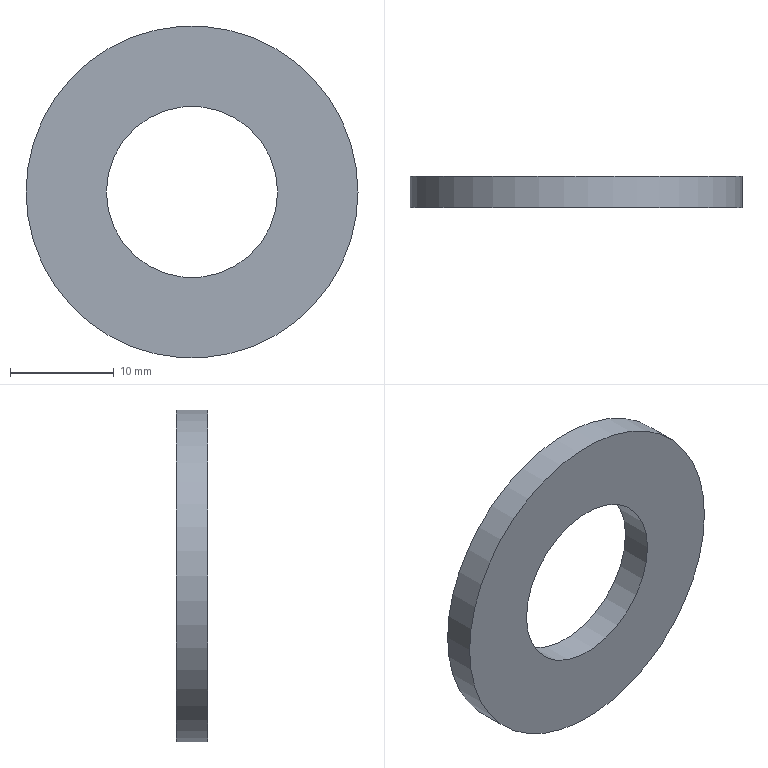Component | NX | WASHER | 1 solid | 4 faces | box 32 x 3 x 32 mm | volume 1771 mm3 | cylinder 2 | plane 2 | commonest cylinder face diameters 32 x1 16.5 x1
STEP:
#1=CARTESIAN_POINT('',(0.,0.,0.));
#2=DIRECTION('',(0.,0.,1.));
#3=DIRECTION('',(1.,0.,0.));
#4=AXIS2_PLACEMENT_3D('',#1,#2,#3);
#5=CARTESIAN_POINT('',(-1.,48.,105.));
#6=VERTEX_POINT('',#5);
#7=CARTESIAN_POINT('',(-17.,48.,105.));
#8=DIRECTION('',(0.,-1.,0.));
#9=DIRECTION('',(1.,0.,0.));
#10=AXIS2_PLACEMENT_3D('',#7,#8,#9);
#11=CIRCLE('',#10,16.);
#12=CARTESIAN_POINT('',(-17.,48.,105.));
#13=DIRECTION('',(0.,-1.,0.));
#14=DIRECTION('',(0.,0.,-1.));
#15=AXIS2_PLACEMENT_3D('',#12,#13,#14);
#16=CYLINDRICAL_SURFACE('',#15,16.);
#17=CARTESIAN_POINT('',(1.571,0.));
#18=DIRECTION('',(1.,0.));
#19=VECTOR('',#18,1.);
#20=LINE('',#17,#19);
#21=(GEOMETRIC_REPRESENTATION_CONTEXT(2)PARAMETRIC_REPRESENTATION_CONTEXT()REPRESENTATION_CONTEXT('',''));
#22=DEFINITIONAL_REPRESENTATION('',(#20),#21);
#23=PCURVE('',#16,#22);
#24=CARTESIAN_POINT('',(-17.,48.,105.));
#25=DIRECTION('',(0.,-1.,0.));
#26=DIRECTION('',(0.,0.,-1.));
#27=AXIS2_PLACEMENT_3D('',#24,#25,#26);
#28=PLANE('',#27);
#29=CARTESIAN_POINT('',(0.,0.));
#30=DIRECTION('',(0.,1.));
#31=AXIS2_PLACEMENT_2D('',#29,#30);
#32=CIRCLE('',#31,16.);
#33=(GEOMETRIC_REPRESENTATION_CONTEXT(2)PARAMETRIC_REPRESENTATION_CONTEXT()REPRESENTATION_CONTEXT('',''));
#34=DEFINITIONAL_REPRESENTATION('',(#32),#33);
#35=PCURVE('',#28,#34);
#36=SURFACE_CURVE('',#11,(#23,#35),.PCURVE_S1.);
#37=EDGE_CURVE('',#6,#6,#36,.T.);
#38=ORIENTED_EDGE('',*,*,#37,.T.);
#39=CARTESIAN_POINT('',(-1.,45.,105.));
#40=VERTEX_POINT('',#39);
#41=CARTESIAN_POINT('',(-1.,48.,105.));
#42=CARTESIAN_POINT('',(-1.,45.,105.));
#43=B_SPLINE_CURVE_WITH_KNOTS('',1,(#41,#42),.UNSPECIFIED.,.F.,.F.,(2,2),(0.,3.),.PIECEWISE_BEZIER_KNOTS.);
#44=CARTESIAN_POINT('',(7.854,0.));
#45=DIRECTION('',(0.,1.));
#46=VECTOR('',#45,1.);
#47=LINE('',#44,#46);
#48=(GEOMETRIC_REPRESENTATION_CONTEXT(2)PARAMETRIC_REPRESENTATION_CONTEXT()REPRESENTATION_CONTEXT('',''));
#49=DEFINITIONAL_REPRESENTATION('',(#47),#48);
#50=PCURVE('',#16,#49);
#51=CARTESIAN_POINT('',(1.571,0.));
#52=DIRECTION('',(0.,1.));
#53=VECTOR('',#52,1.);
#54=LINE('',#51,#53);
#55=(GEOMETRIC_REPRESENTATION_CONTEXT(2)PARAMETRIC_REPRESENTATION_CONTEXT()REPRESENTATION_CONTEXT('',''));
#56=DEFINITIONAL_REPRESENTATION('',(#54),#55);
#57=PCURVE('',#16,#56);
#58=SEAM_CURVE('',#43,(#50,#57),.PCURVE_S1.);
#59=EDGE_CURVE('',#6,#40,#58,.T.);
#60=ORIENTED_EDGE('',*,*,#59,.T.);
#61=CARTESIAN_POINT('',(-17.,45.,105.));
#62=DIRECTION('',(0.,-1.,0.));
#63=DIRECTION('',(1.,0.,0.));
#64=AXIS2_PLACEMENT_3D('',#61,#62,#63);
#65=CIRCLE('',#64,16.);
#66=CARTESIAN_POINT('',(1.571,3.));
#67=DIRECTION('',(1.,0.));
#68=VECTOR('',#67,1.);
#69=LINE('',#66,#68);
#70=(GEOMETRIC_REPRESENTATION_CONTEXT(2)PARAMETRIC_REPRESENTATION_CONTEXT()REPRESENTATION_CONTEXT('',''));
#71=DEFINITIONAL_REPRESENTATION('',(#69),#70);
#72=PCURVE('',#16,#71);
#73=CARTESIAN_POINT('',(-17.,45.,105.));
#74=DIRECTION('',(0.,-1.,0.));
#75=DIRECTION('',(0.,0.,-1.));
#76=AXIS2_PLACEMENT_3D('',#73,#74,#75);
#77=PLANE('',#76);
#78=CARTESIAN_POINT('',(0.,0.));
#79=DIRECTION('',(0.,1.));
#80=AXIS2_PLACEMENT_2D('',#78,#79);
#81=CIRCLE('',#80,16.);
#82=(GEOMETRIC_REPRESENTATION_CONTEXT(2)PARAMETRIC_REPRESENTATION_CONTEXT()REPRESENTATION_CONTEXT('',''));
#83=DEFINITIONAL_REPRESENTATION('',(#81),#82);
#84=PCURVE('',#77,#83);
#85=SURFACE_CURVE('',#65,(#72,#84),.PCURVE_S1.);
#86=EDGE_CURVE('',#40,#40,#85,.T.);
#87=ORIENTED_EDGE('',*,*,#86,.F.);
#88=ORIENTED_EDGE('',*,*,#59,.F.);
#89=EDGE_LOOP('',(#38,#60,#87,#88));
#90=FACE_BOUND('',#89,.T.);
#91=ADVANCED_FACE('',(#90),#16,.T.);
#92=CARTESIAN_POINT('',(-8.75,48.,105.));
#93=VERTEX_POINT('',#92);
#94=CARTESIAN_POINT('',(-17.,48.,105.));
#95=DIRECTION('',(0.,-1.,0.));
#96=DIRECTION('',(1.,0.,0.));
#97=AXIS2_PLACEMENT_3D('',#94,#95,#96);
#98=CIRCLE('',#97,8.25);
#99=CARTESIAN_POINT('',(-17.,48.,105.));
#100=DIRECTION('',(0.,-1.,0.));
#101=DIRECTION('',(0.,0.,-1.));
#102=AXIS2_PLACEMENT_3D('',#99,#100,#101);
#103=CYLINDRICAL_SURFACE('',#102,8.25);
#104=CARTESIAN_POINT('',(1.571,0.));
#105=DIRECTION('',(1.,0.));
#106=VECTOR('',#105,1.);
#107=LINE('',#104,#106);
#108=(GEOMETRIC_REPRESENTATION_CONTEXT(2)PARAMETRIC_REPRESENTATION_CONTEXT()REPRESENTATION_CONTEXT('',''));
#109=DEFINITIONAL_REPRESENTATION('',(#107),#108);
#110=PCURVE('',#103,#109);
#111=CARTESIAN_POINT('',(0.,0.));
#112=DIRECTION('',(0.,1.));
#113=AXIS2_PLACEMENT_2D('',#111,#112);
#114=CIRCLE('',#113,8.25);
#115=(GEOMETRIC_REPRESENTATION_CONTEXT(2)PARAMETRIC_REPRESENTATION_CONTEXT()REPRESENTATION_CONTEXT('',''));
#116=DEFINITIONAL_REPRESENTATION('',(#114),#115);
#117=PCURVE('',#28,#116);
#118=SURFACE_CURVE('',#98,(#110,#117),.PCURVE_S1.);
#119=EDGE_CURVE('',#93,#93,#118,.T.);
#120=ORIENTED_EDGE('',*,*,#119,.T.);
#121=CARTESIAN_POINT('',(-8.75,45.,105.));
#122=VERTEX_POINT('',#121);
#123=CARTESIAN_POINT('',(-8.75,48.,105.));
#124=CARTESIAN_POINT('',(-8.75,45.,105.));
#125=B_SPLINE_CURVE_WITH_KNOTS('',1,(#123,#124),.UNSPECIFIED.,.F.,.F.,(2,2),(0.,3.),.PIECEWISE_BEZIER_KNOTS.);
#126=CARTESIAN_POINT('',(7.854,0.));
#127=DIRECTION('',(0.,1.));
#128=VECTOR('',#127,1.);
#129=LINE('',#126,#128);
#130=(GEOMETRIC_REPRESENTATION_CONTEXT(2)PARAMETRIC_REPRESENTATION_CONTEXT()REPRESENTATION_CONTEXT('',''));
#131=DEFINITIONAL_REPRESENTATION('',(#129),#130);
#132=PCURVE('',#103,#131);
#133=CARTESIAN_POINT('',(1.571,0.));
#134=DIRECTION('',(0.,1.));
#135=VECTOR('',#134,1.);
#136=LINE('',#133,#135);
#137=(GEOMETRIC_REPRESENTATION_CONTEXT(2)PARAMETRIC_REPRESENTATION_CONTEXT()REPRESENTATION_CONTEXT('',''));
#138=DEFINITIONAL_REPRESENTATION('',(#136),#137);
#139=PCURVE('',#103,#138);
#140=SEAM_CURVE('',#125,(#132,#139),.PCURVE_S1.);
#141=EDGE_CURVE('',#93,#122,#140,.T.);
#142=ORIENTED_EDGE('',*,*,#141,.T.);
#143=CARTESIAN_POINT('',(-17.,45.,105.));
#144=DIRECTION('',(0.,-1.,0.));
#145=DIRECTION('',(1.,0.,0.));
#146=AXIS2_PLACEMENT_3D('',#143,#144,#145);
#147=CIRCLE('',#146,8.25);
#148=CARTESIAN_POINT('',(1.571,3.));
#149=DIRECTION('',(1.,0.));
#150=VECTOR('',#149,1.);
#151=LINE('',#148,#150);
#152=(GEOMETRIC_REPRESENTATION_CONTEXT(2)PARAMETRIC_REPRESENTATION_CONTEXT()REPRESENTATION_CONTEXT('',''));
#153=DEFINITIONAL_REPRESENTATION('',(#151),#152);
#154=PCURVE('',#103,#153);
#155=CARTESIAN_POINT('',(0.,0.));
#156=DIRECTION('',(0.,1.));
#157=AXIS2_PLACEMENT_2D('',#155,#156);
#158=CIRCLE('',#157,8.25);
#159=(GEOMETRIC_REPRESENTATION_CONTEXT(2)PARAMETRIC_REPRESENTATION_CONTEXT()REPRESENTATION_CONTEXT('',''));
#160=DEFINITIONAL_REPRESENTATION('',(#158),#159);
#161=PCURVE('',#77,#160);
#162=SURFACE_CURVE('',#147,(#154,#161),.PCURVE_S1.);
#163=EDGE_CURVE('',#122,#122,#162,.T.);
#164=ORIENTED_EDGE('',*,*,#163,.F.);
#165=ORIENTED_EDGE('',*,*,#141,.F.);
#166=EDGE_LOOP('',(#120,#142,#164,#165));
#167=FACE_BOUND('',#166,.F.);
#168=ADVANCED_FACE('',(#167),#103,.F.);
#169=ORIENTED_EDGE('',*,*,#37,.F.);
#170=EDGE_LOOP('',(#169));
#171=FACE_BOUND('',#170,.T.);
#172=ORIENTED_EDGE('',*,*,#119,.T.);
#173=EDGE_LOOP('',(#172));
#174=FACE_BOUND('',#173,.T.);
#175=ADVANCED_FACE('',(#171,#174),#28,.F.);
#176=ORIENTED_EDGE('',*,*,#86,.T.);
#177=EDGE_LOOP('',(#176));
#178=FACE_BOUND('',#177,.T.);
#179=ORIENTED_EDGE('',*,*,#163,.F.);
#180=EDGE_LOOP('',(#179));
#181=FACE_BOUND('',#180,.T.);
#182=ADVANCED_FACE('',(#178,#181),#77,.T.);
#183=CLOSED_SHELL('',(#91,#168,#175,#182));
#184=MANIFOLD_SOLID_BREP('',#183);
#185=(LENGTH_UNIT()NAMED_UNIT(*)SI_UNIT(.MILLI.,.METRE.));
#186=UNCERTAINTY_MEASURE_WITH_UNIT(LENGTH_MEASURE(0.00001),#185,'','');
#187=(NAMED_UNIT(*)PLANE_ANGLE_UNIT()SI_UNIT($,.RADIAN.));
#188=(NAMED_UNIT(*)SI_UNIT($,.STERADIAN.)SOLID_ANGLE_UNIT());
#189=(GEOMETRIC_REPRESENTATION_CONTEXT(3)GLOBAL_UNCERTAINTY_ASSIGNED_CONTEXT((#186))GLOBAL_UNIT_ASSIGNED_CONTEXT((#185,#187,#188))REPRESENTATION_CONTEXT('',''));
#190=ADVANCED_BREP_SHAPE_REPRESENTATION('',(#4,#184),#189);